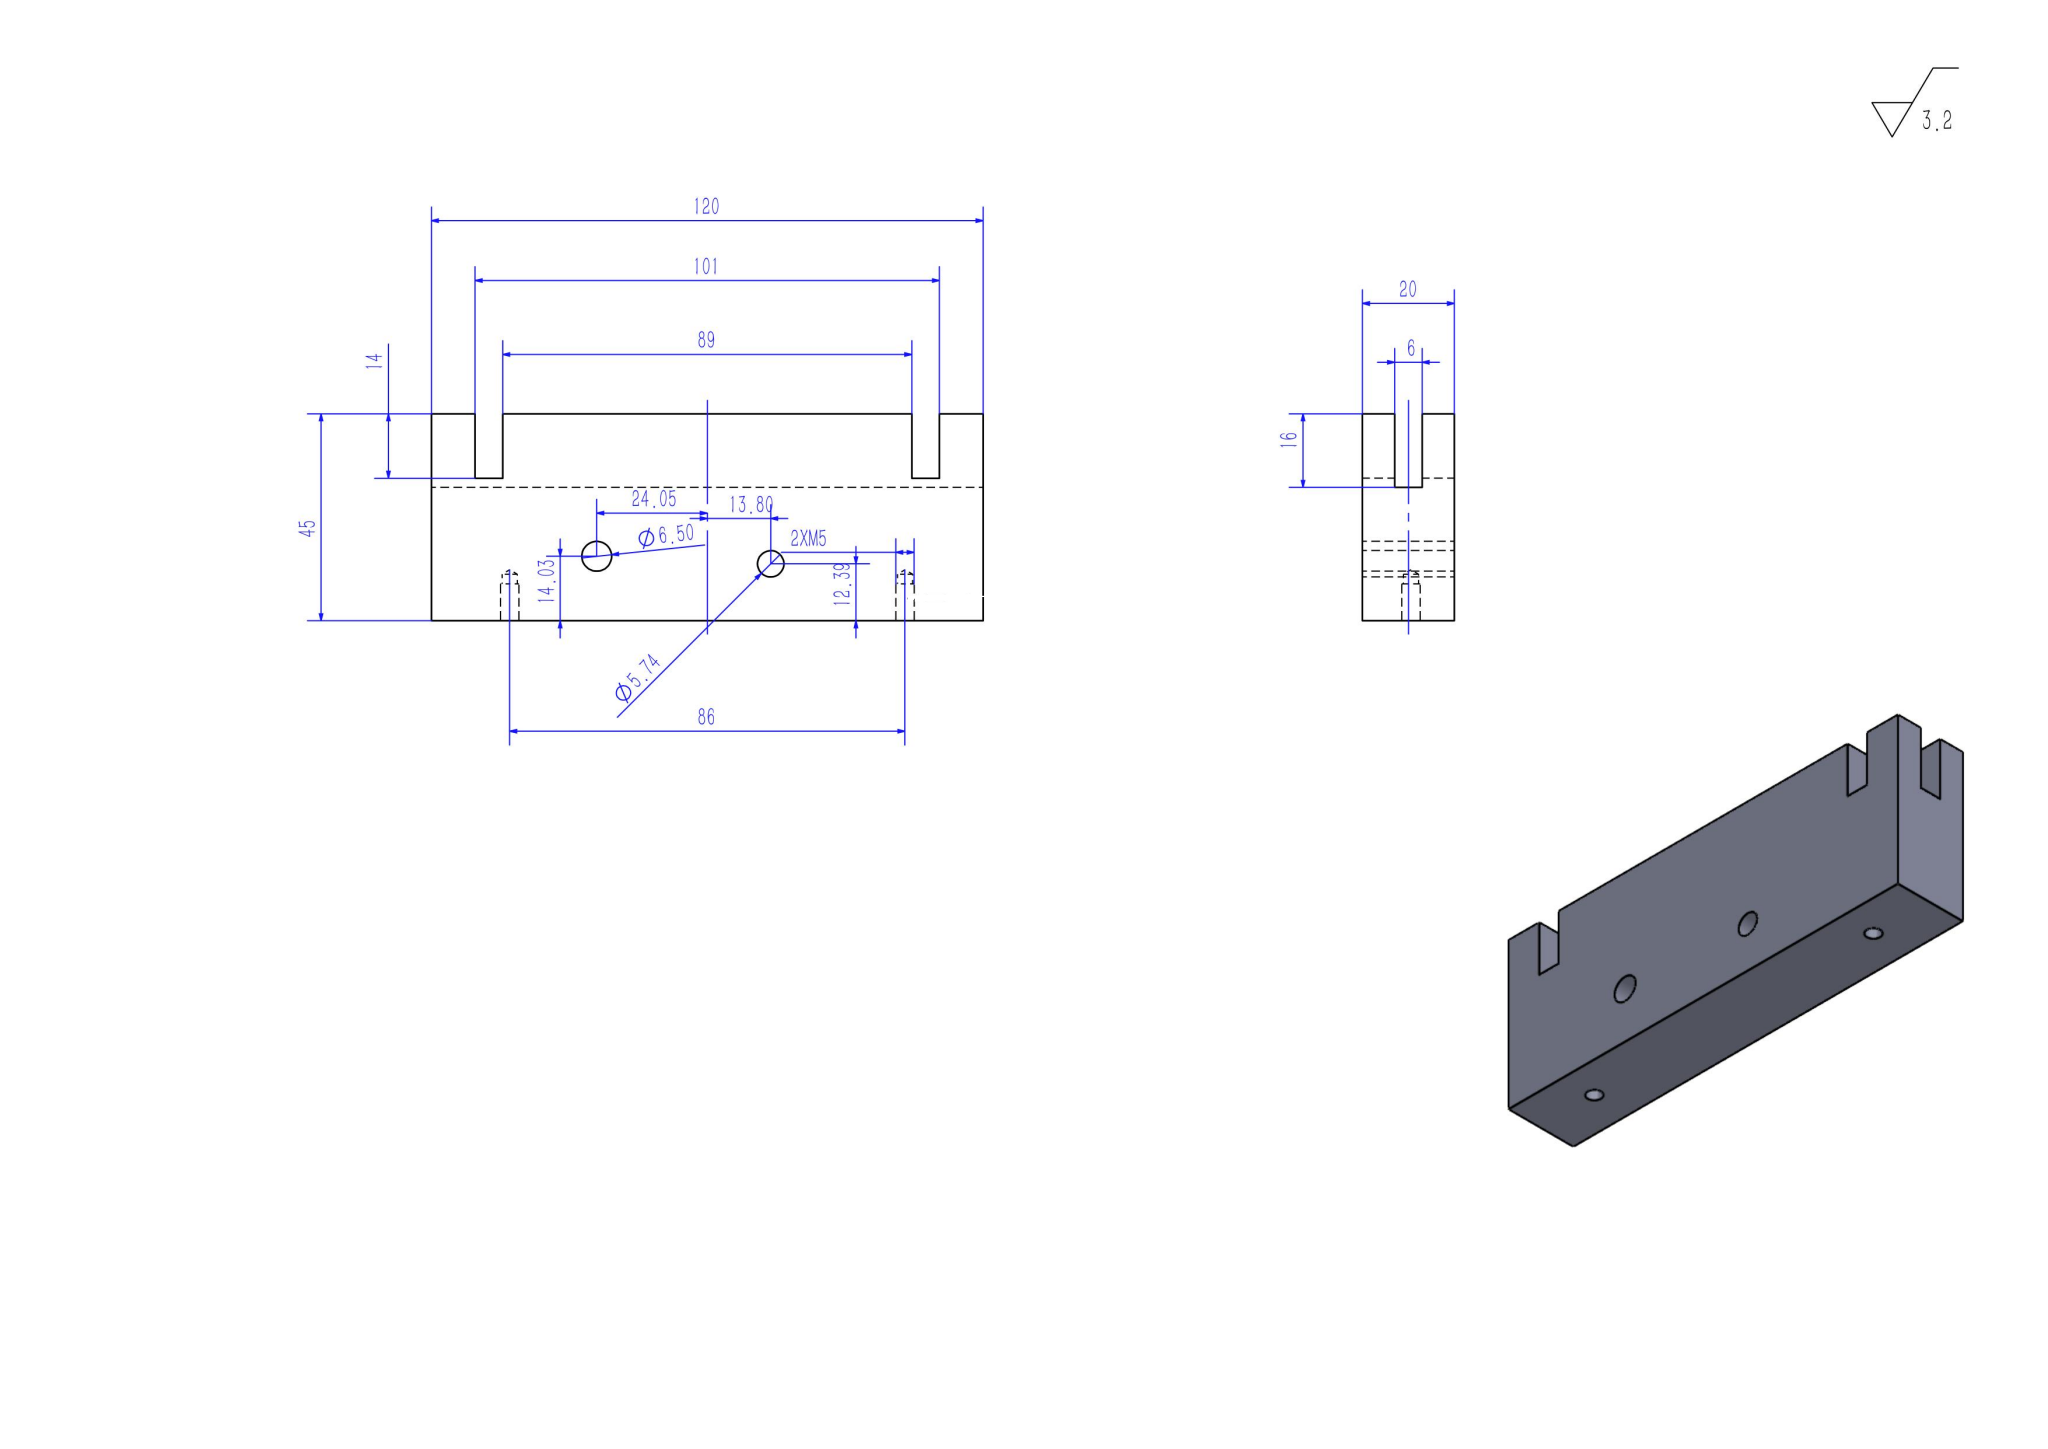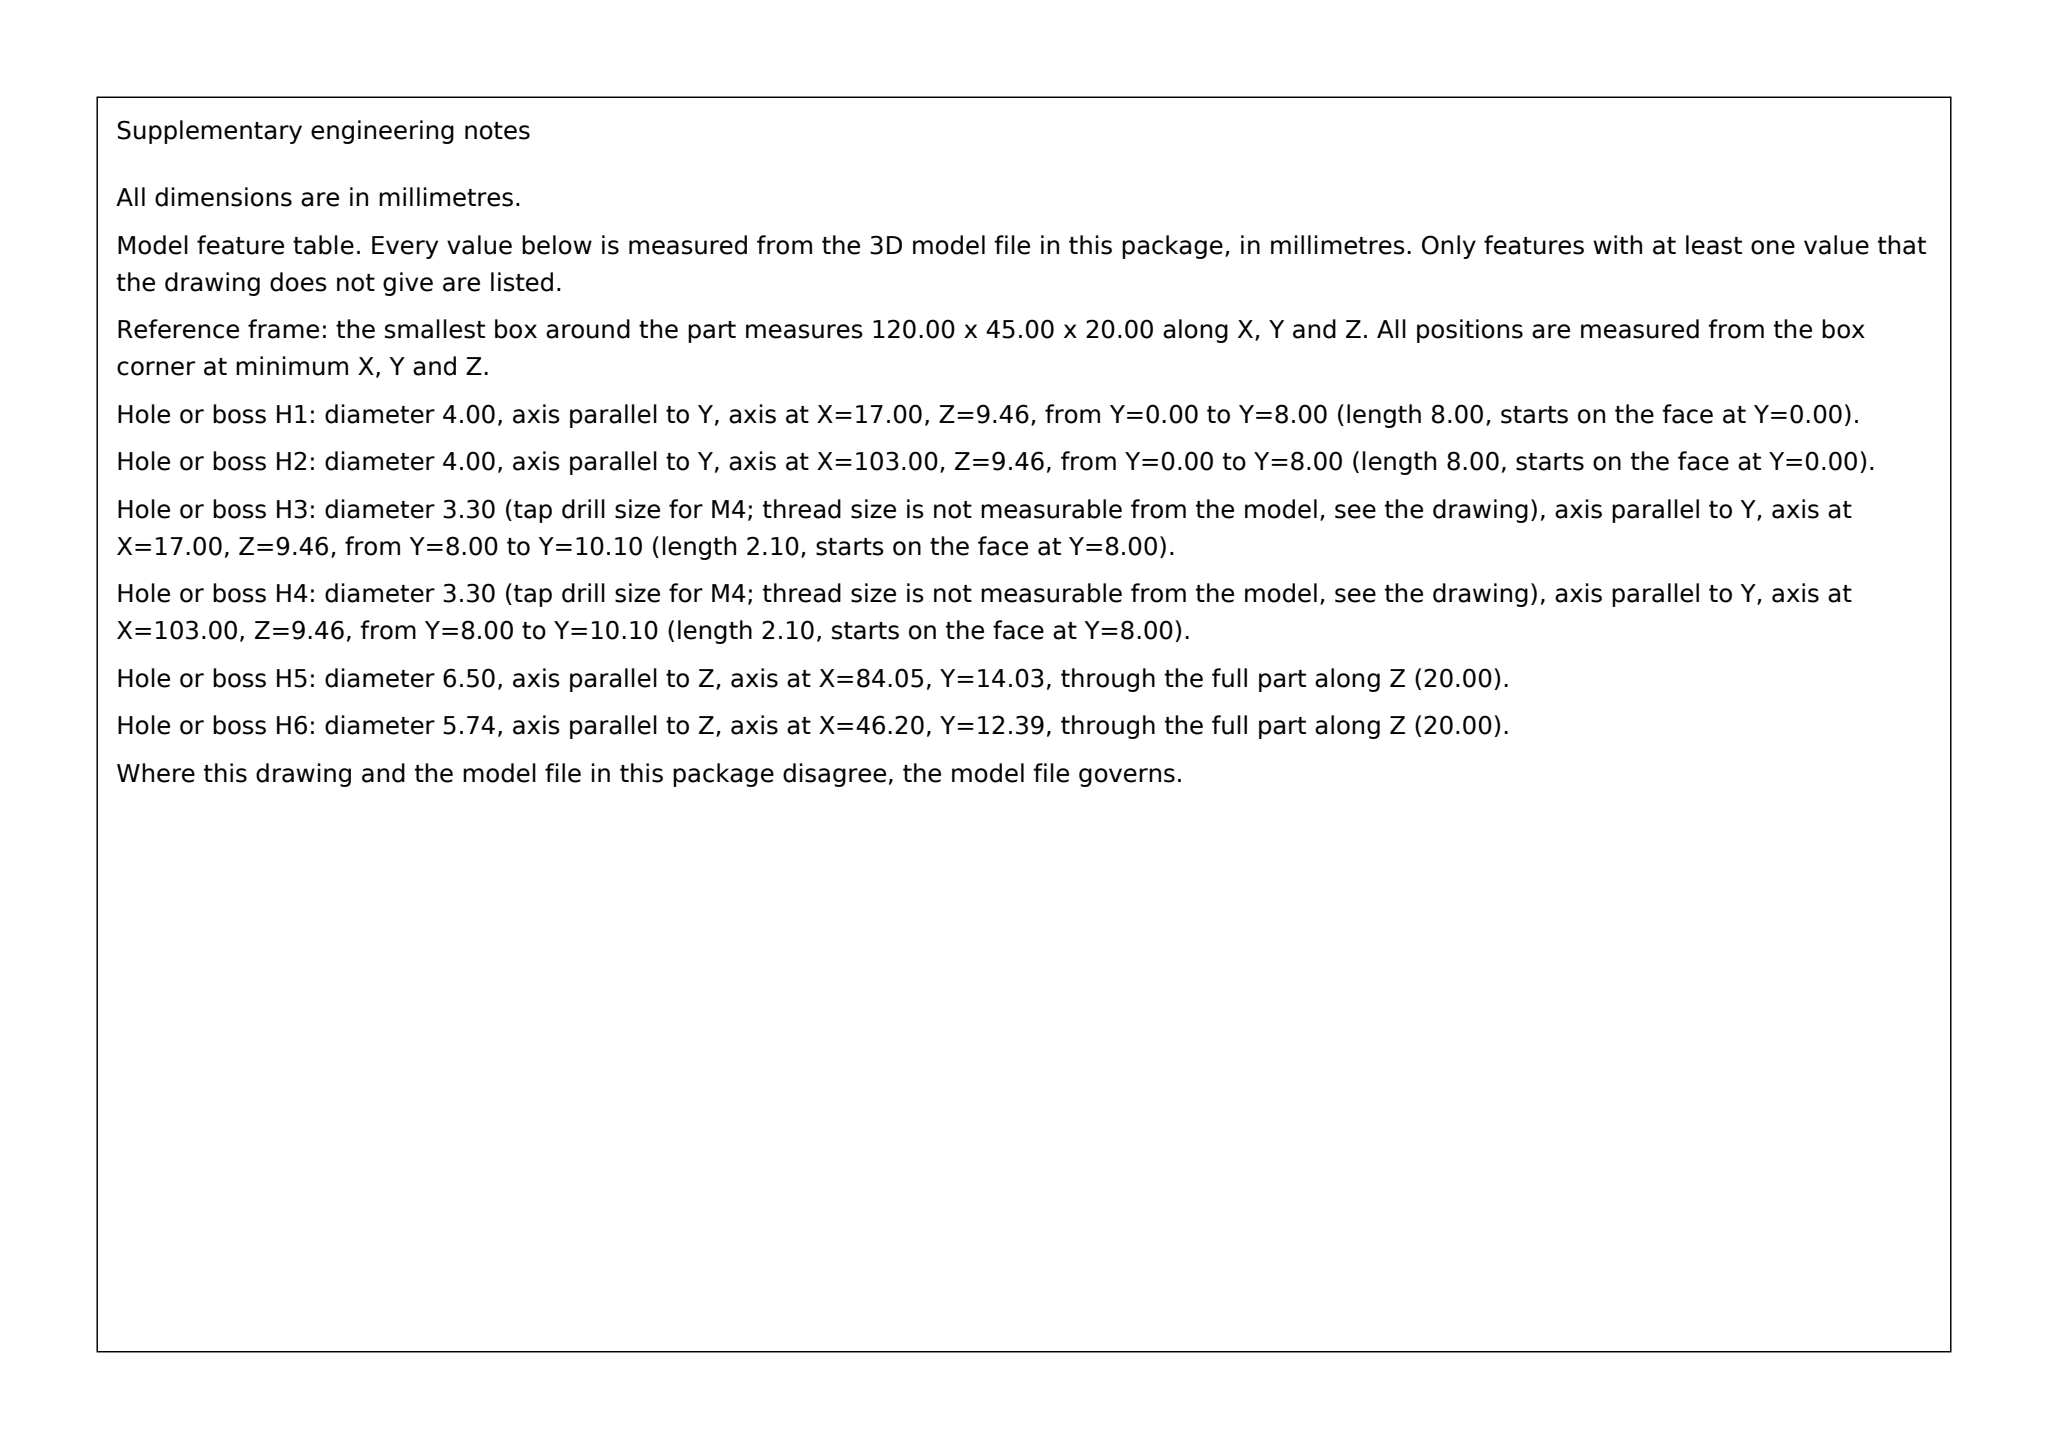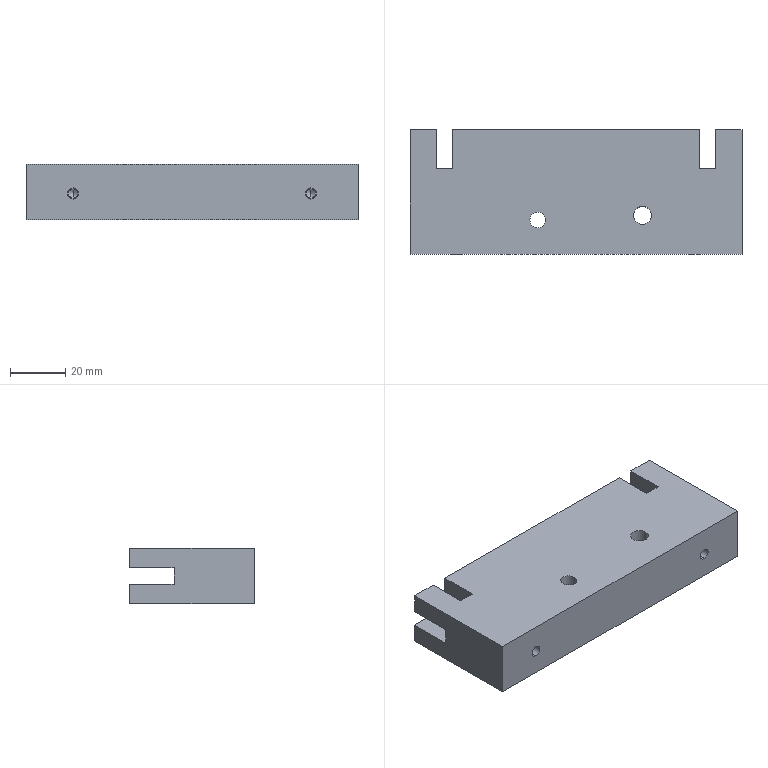Part | SolidWorks | mm | 1 solid | 44 faces | box 120 x 45 x 20 mm | volume 92705 mm3 | plane 28 | cylinder 12 | cone 4 | commonest cylinder face diameters 4 x4 3.3 x4 5.738 x2 6.495 x2
build123d program:
from build123d import *

# Parameters (mm, degrees)
SKETCH1_W                   = 20
SKETCH1_H                   = 45
BOSS_EXTRUDE1_DEPTH         = 60
CUT_EXTRUDE1_DEPTH          = 123.5
SKETCH3_W                   = 6
SKETCH3_H                   = 20.21
CUT_EXTRUDE2_DEPTH          = 120
M4_TAPPED_HOLE1_D           = 3.3
M4_TAPPED_HOLE1_DEPTH       = 10.1
M4_TAPPED_HOLE1_CBORE_D     = 4
M4_TAPPED_HOLE1_CBORE_DEPTH = 8
M4_TAPPED_HOLE1_TIP         = 0.9914
SKETCH10_R                  = 2.869
SKETCH10_R_2                = 3.248
CUT_EXTRUDE3_DEPTH          = 80


with BuildPart() as part:
    # Sketch1 → Boss-Extrude1 (new, symmetric)
    with BuildSketch(Plane(origin=(0, 0, 0), x_dir=(0, 0, -1), z_dir=(1, 0, 0))):
        Rectangle(SKETCH1_W, SKETCH1_H)
    extrude(amount=BOSS_EXTRUDE1_DEPTH, both=True)

    # Sketch2 → Cut-Extrude1 (cut, through all)
    with BuildSketch(Plane(origin=(60, 0, 0), x_dir=(0, 0, -1), z_dir=(1, 0, 0))):
        with BuildLine():
            Line((-3, 6.5), (-3, 24.876))
            ThreePointArc((-3, 24.876), (-0.00001561, 70.823), (3, 24.876))
            Line((3, 24.876), (3, 6.5))
            Line((3, 6.5), (-3, 6.5))
        make_face()
    extrude(amount=-CUT_EXTRUDE1_DEPTH, mode=Mode.SUBTRACT)

    # Sketch3 → Cut-Extrude2 (cut)
    with BuildSketch(Plane(origin=(0, 0, -10), x_dir=(-1, 0, 0), z_dir=(0, 0, -1))):
        with Locations((-47.5, 18.605)):
            Rectangle(SKETCH3_W, SKETCH3_H)
        with Locations((47.5, 18.605)):
            Rectangle(SKETCH3_W, SKETCH3_H)
    extrude(amount=-CUT_EXTRUDE2_DEPTH, mode=Mode.SUBTRACT)

    # M4 Tapped Hole1
    with Locations(Plane(origin=(0, -22.5, 0), x_dir=(-1, 0, 0), z_dir=(0, -1, 0))):
        with Locations((43, 0.5397), (-43, 0.5397)):
            CounterBoreHole(M4_TAPPED_HOLE1_D / 2, M4_TAPPED_HOLE1_CBORE_D / 2, M4_TAPPED_HOLE1_CBORE_DEPTH, depth=M4_TAPPED_HOLE1_DEPTH)
            with Locations((0, 0, -(M4_TAPPED_HOLE1_DEPTH + M4_TAPPED_HOLE1_TIP / 2))):  # 118° drill point
                Cone(0, M4_TAPPED_HOLE1_D / 2, M4_TAPPED_HOLE1_TIP, mode=Mode.SUBTRACT)

    # Sketch10 → Cut-Extrude3 (cut)
    with BuildSketch(Plane.XY.offset(10)):
        with Locations((-13.799, -10.11)):
            Circle(SKETCH10_R)
        with Locations((24.046, -8.471)):
            Circle(SKETCH10_R_2)
    extrude(amount=-CUT_EXTRUDE3_DEPTH, mode=Mode.SUBTRACT)


solid = part.part